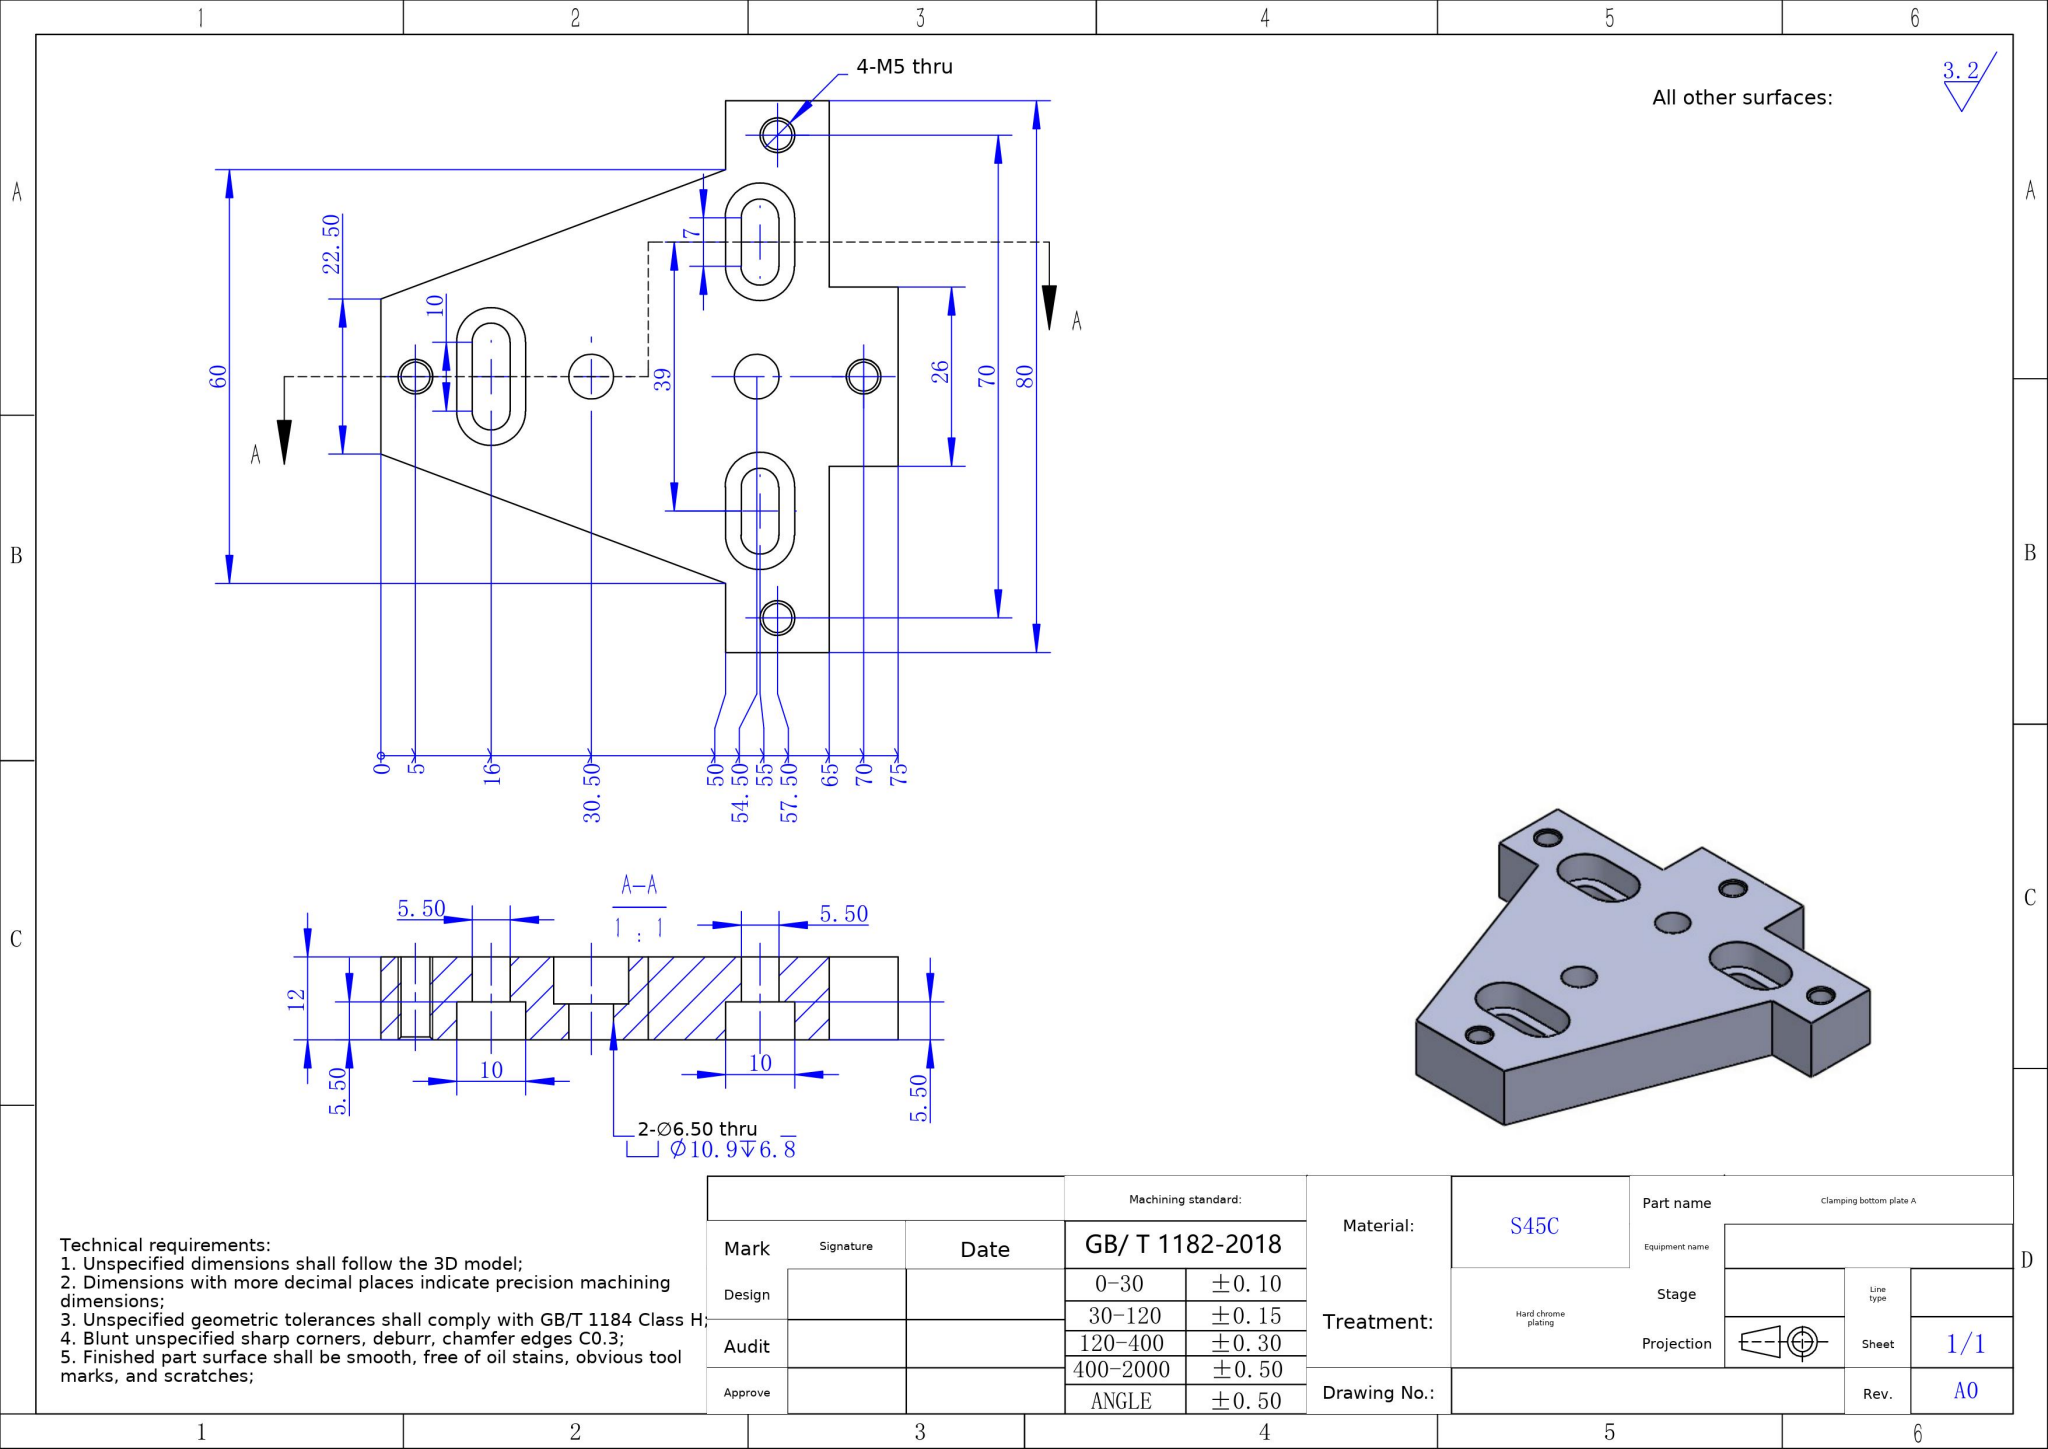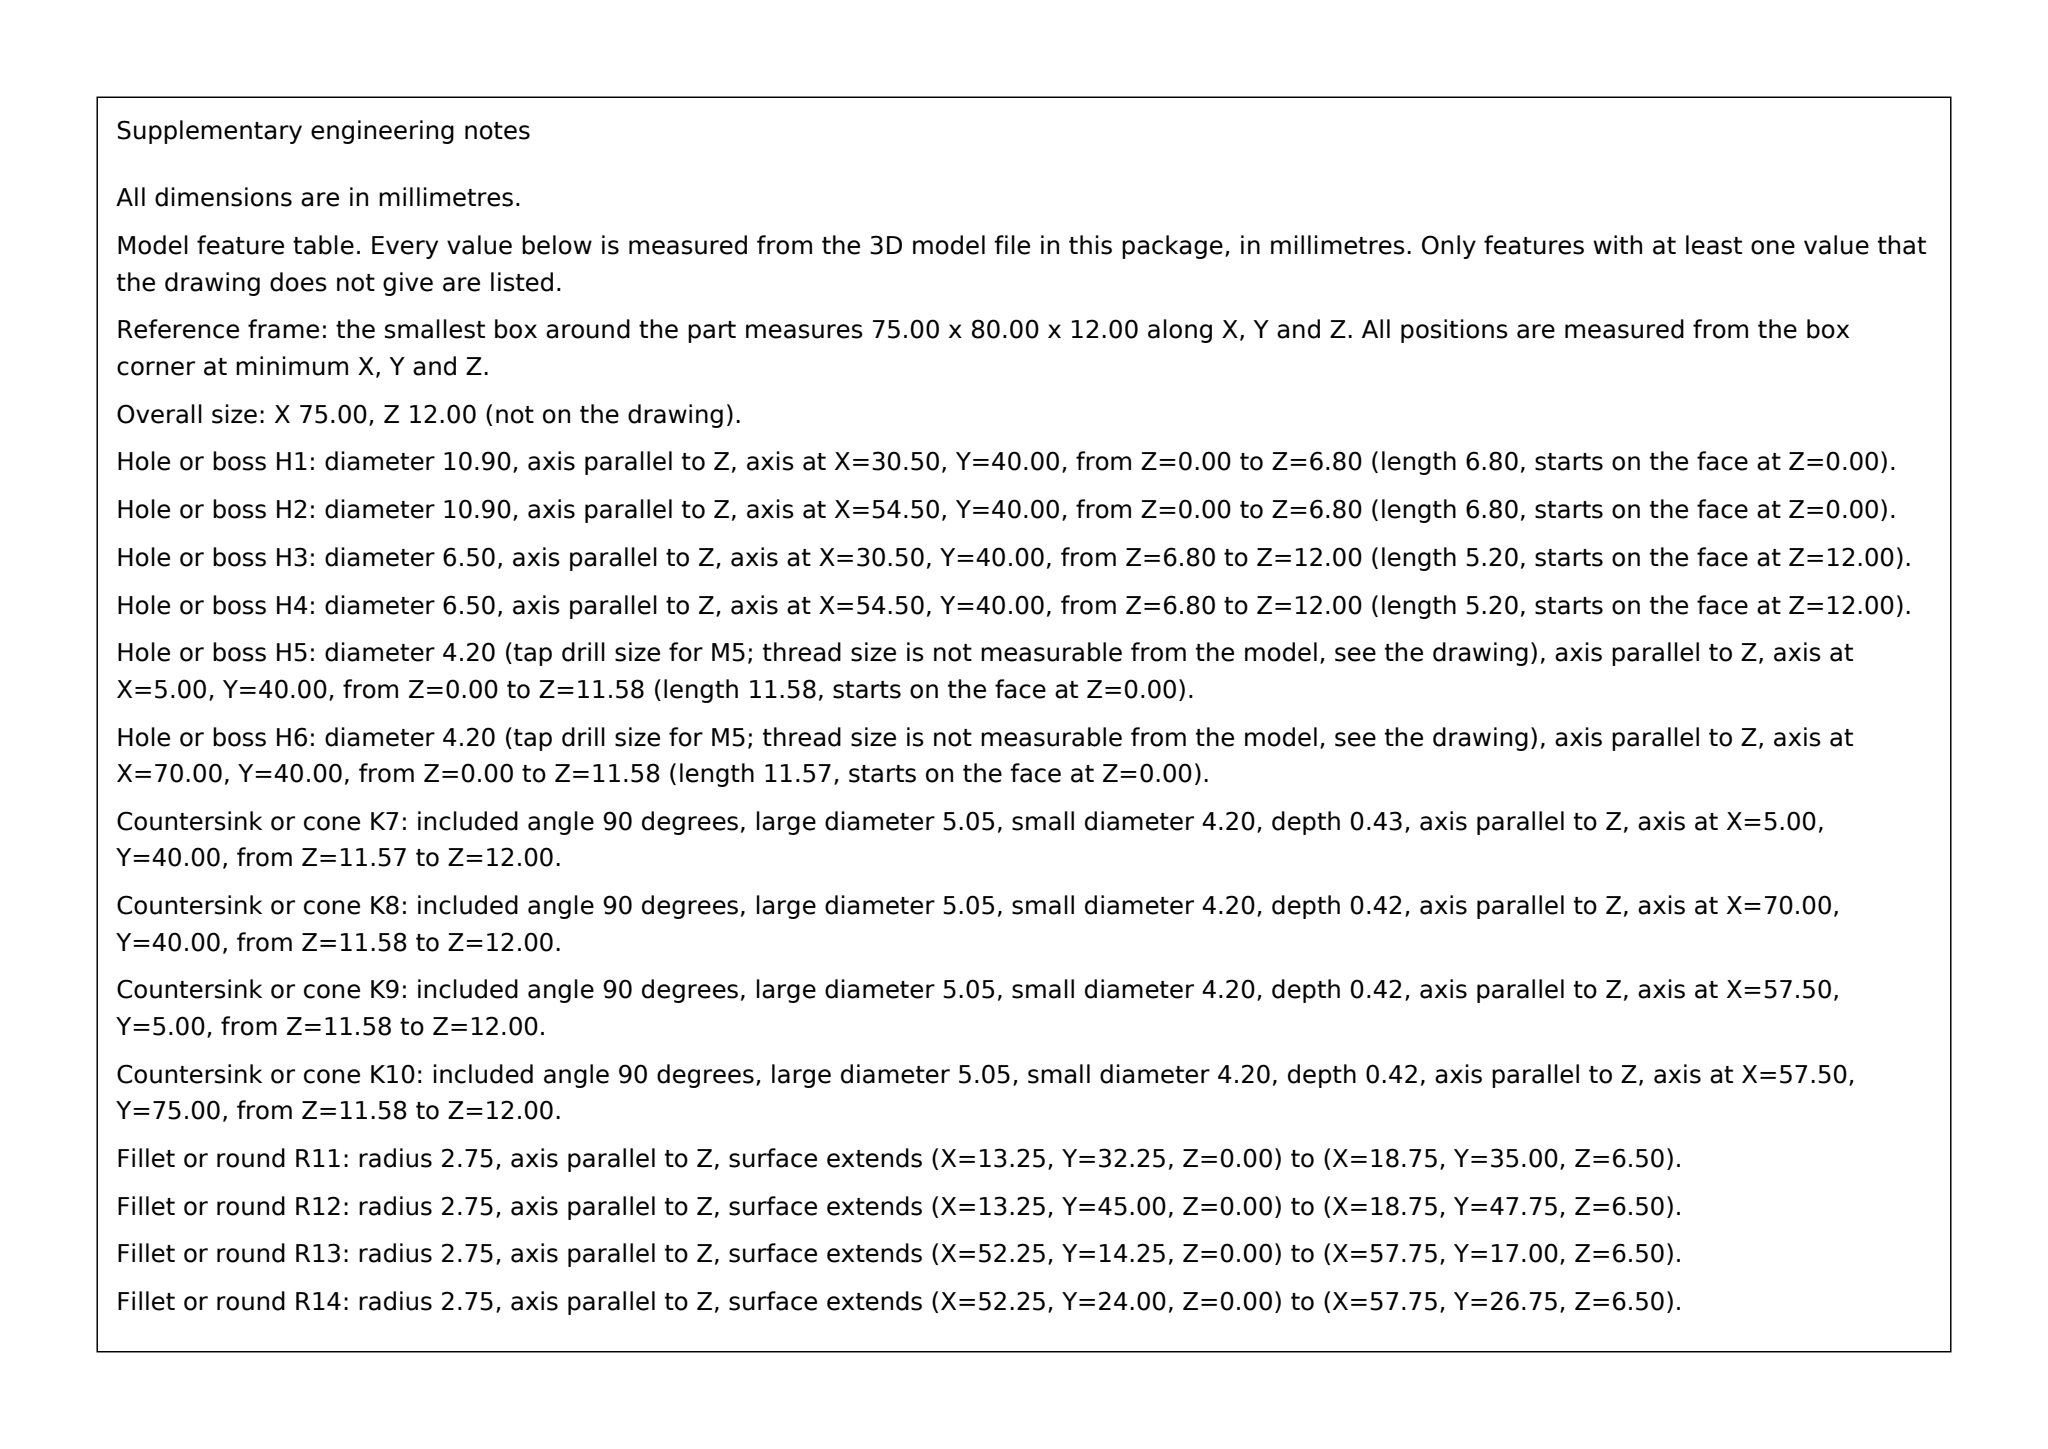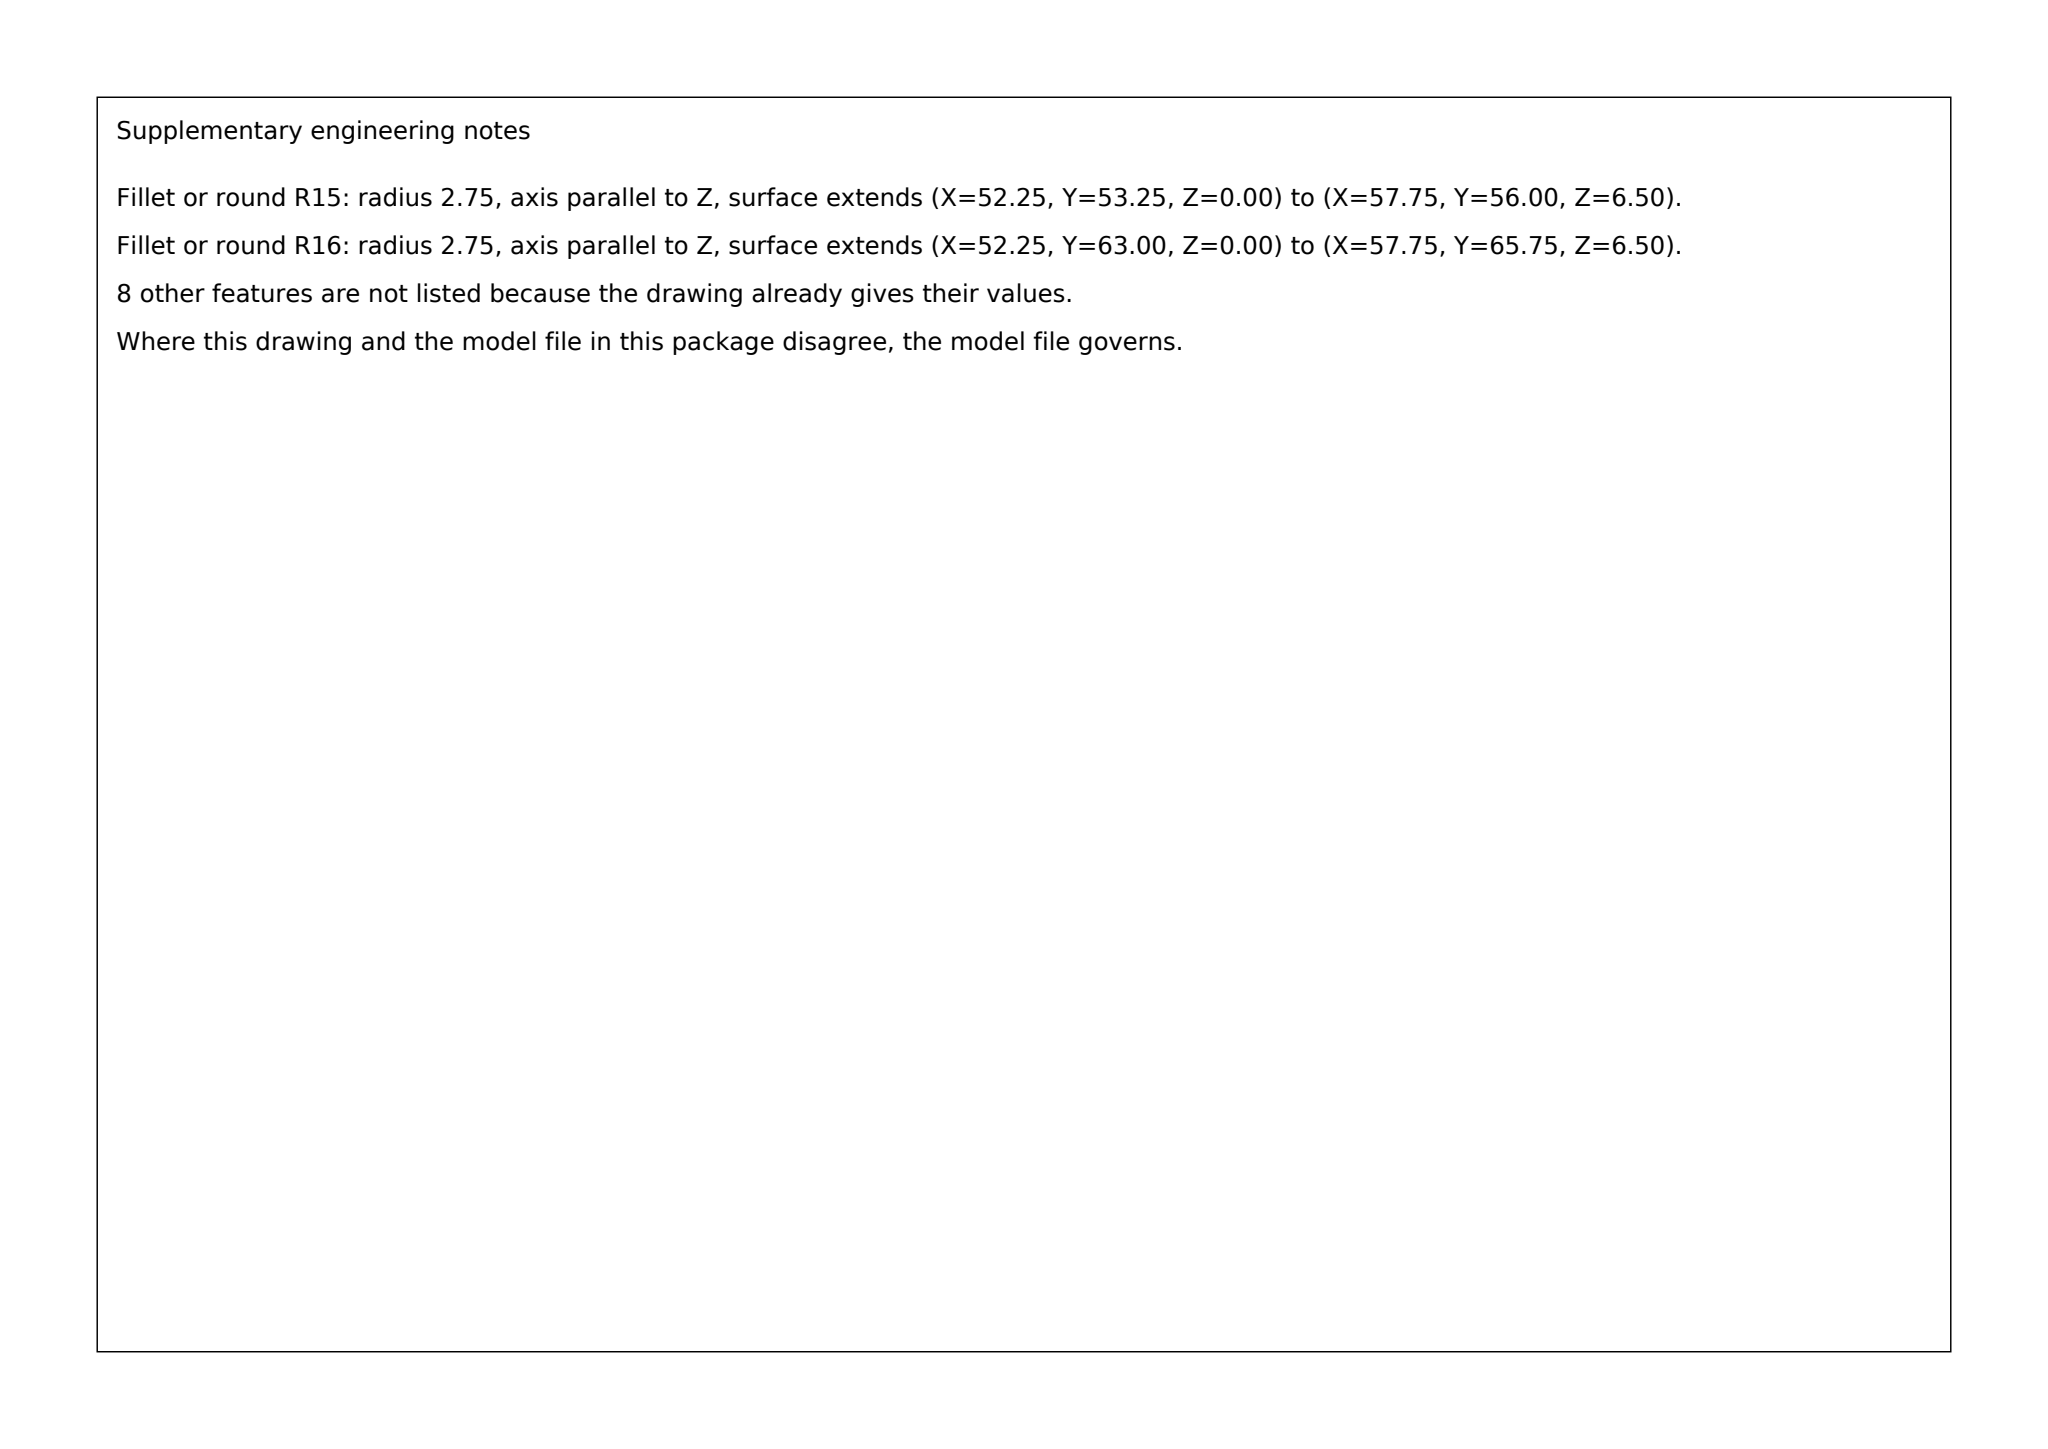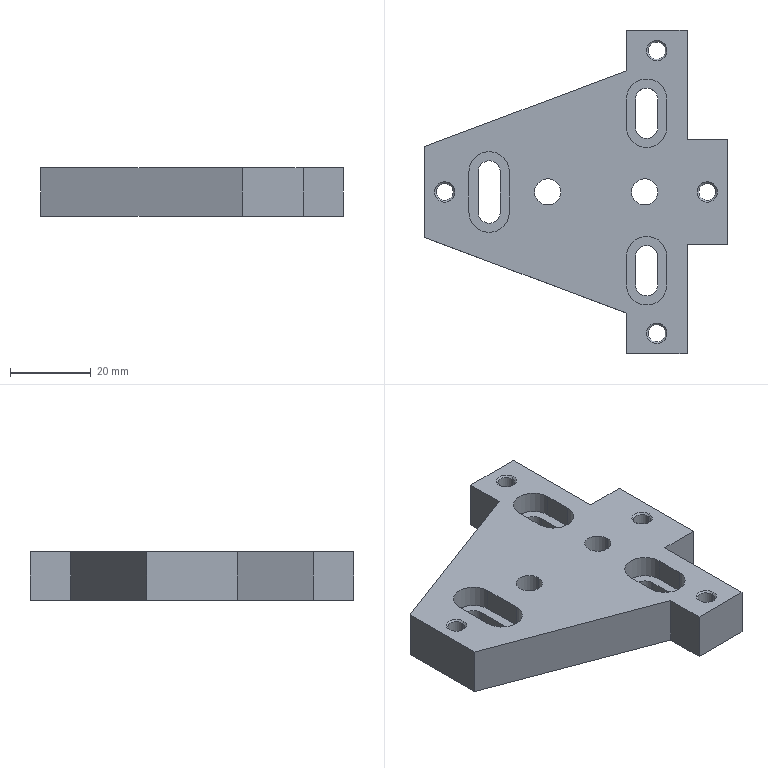Part | SolidWorks | mm | material S45C | 1 solid | 67 faces | box 75 x 80 x 12 mm | volume 36049 mm3 | plane 31 | cylinder 28 | cone 8 | commonest cylinder face diameters 4.2 x8 5.5 x6 10 x6 10.9 x4 6.5 x4
build123d program:
from build123d import *

# Parameters (mm, degrees)
BOSS_EXTRUDE1_DEPTH         = 12
CUT_EXTRUDE1_DEPTH          = 64.789
CUT_EXTRUDE2_DEPTH          = 5.5
SKETCH4_R                   = 3.25
CUT_EXTRUDE3_DEPTH          = 64.789
SKETCH5_W                   = 10
SKETCH5_H                   = 30
SKETCH5_W_2                 = 15
SKETCH5_H_2                 = 10
BOSS_EXTRUDE2_DEPTH         = 12
M5_TAPPED_HOLE1_D           = 4.2
M5_TAPPED_HOLE1_CSINK_D     = 5.05
M5_TAPPED_HOLE1_CSINK_ANGLE = 90
CUT_EXTRUDE4_DEPTH          = 78.259
SKETCH9_W                   = 10
SKETCH9_H                   = 26
BOSS_EXTRUDE3_DEPTH         = 12
M5_TAPPED_HOLE2_D           = 4.2
M5_TAPPED_HOLE2_CSINK_D     = 5.05
M5_TAPPED_HOLE2_CSINK_ANGLE = 90
SKETCH12_R                  = 5.45
CUT_EXTRUDE5_DEPTH          = 6.8


with BuildPart() as part:
    # Sketch1 → Boss-Extrude1 (new body)
    with BuildSketch(Plane.XY):
        Polygon((0, -30), (0, 30), (-15, 30), (-55, 15), (-55, -15), (-15, -30), align=None)
    extrude(amount=BOSS_EXTRUDE1_DEPTH)

    # Sketch2 → Cut-Extrude1 (cut, through all)
    with BuildSketch(Plane.XY.offset(12)):
        with BuildLine():
            Line((-46.25, 5), (-46.25, -5))
            ThreePointArc((-46.25, -5), (-49, -7.75), (-51.75, -5))
            Line((-51.75, -5), (-51.75, 5))
            ThreePointArc((-51.75, 5), (-49, 7.75), (-46.25, 5))
        make_face()
        with BuildLine():
            Line((-7.25, 23), (-7.25, 16))
            ThreePointArc((-7.25, 16), (-10, 13.25), (-12.75, 16))
            Line((-12.75, 16), (-12.75, 23))
            ThreePointArc((-12.75, 23), (-10, 25.75), (-7.25, 23))
        make_face()
        with BuildLine():
            Line((-7.25, -23), (-7.25, -16))
            ThreePointArc((-7.25, -16), (-10, -13.25), (-12.75, -16))
            Line((-12.75, -16), (-12.75, -23))
            ThreePointArc((-12.75, -23), (-10, -25.75), (-7.25, -23))
        make_face()
    extrude(amount=-CUT_EXTRUDE1_DEPTH, mode=Mode.SUBTRACT)

    # Sketch3 → Cut-Extrude2 (cut)
    with BuildSketch(Plane.XY.offset(12)):
        with BuildLine():
            Line((-44, -5), (-44, 5))
            ThreePointArc((-44, 5), (-49, 10), (-54, 5))
            Line((-54, 5), (-54, -5))
            ThreePointArc((-54, -5), (-49, -10), (-44, -5))
        make_face()
        with BuildLine():
            Line((-5, -23), (-5, -16))
            ThreePointArc((-5, -16), (-10, -11), (-15, -16))
            Line((-15, -16), (-15, -23))
            ThreePointArc((-15, -23), (-10, -28), (-5, -23))
        make_face()
        with BuildLine():
            Line((-5, 16), (-5, 23))
            ThreePointArc((-5, 23), (-10, 28), (-15, 23))
            Line((-15, 23), (-15, 16))
            ThreePointArc((-15, 16), (-10, 11), (-5, 16))
        make_face()
    extrude(amount=-CUT_EXTRUDE2_DEPTH, mode=Mode.SUBTRACT)

    # Sketch4 → Cut-Extrude3 (cut, through all)
    with BuildSketch(Plane.XY.offset(12)):
        with Locations((-34.5, 0)):
            Circle(SKETCH4_R)
        with Locations((-10.5, 0)):
            Circle(SKETCH4_R)
    extrude(amount=-CUT_EXTRUDE3_DEPTH, mode=Mode.SUBTRACT)

    # Sketch5 → Boss-Extrude2 (add)
    with BuildSketch(Plane.XY.offset(12)):
        with Locations((-60, 0)):
            Rectangle(SKETCH5_W, SKETCH5_H)
        with Locations((-7.5, 35)):
            Rectangle(SKETCH5_W_2, SKETCH5_H_2)
        with Locations((-7.5, -35)):
            Rectangle(SKETCH5_W_2, SKETCH5_H_2)
    extrude(amount=-BOSS_EXTRUDE2_DEPTH)

    # M5 Tapped Hole1 (through all)
    with Locations(Plane.XY.offset(12)):
        with Locations((-7.5, -35), (-60, 0), (-7.5, 35)):
            CounterSinkHole(M5_TAPPED_HOLE1_D / 2, M5_TAPPED_HOLE1_CSINK_D / 2, counter_sink_angle=M5_TAPPED_HOLE1_CSINK_ANGLE)

    # Sketch8 → Cut-Extrude4 (cut, through all)
    with BuildSketch(Plane.XY.offset(12)):
        Polygon((-55, 15), (-68.605, 22.741), (-66.181, 10.807), align=None)
        Polygon((-68.605, -22.741), (-66.181, -10.807), (-55, -15), align=None)
    extrude(amount=-CUT_EXTRUDE4_DEPTH, mode=Mode.SUBTRACT)

    # Sketch9 → Boss-Extrude3 (add)
    with BuildSketch(Plane.XY.offset(12)):
        with Locations((5, 0)):
            Rectangle(SKETCH9_W, SKETCH9_H)
    extrude(amount=-BOSS_EXTRUDE3_DEPTH)

    # M5 Tapped Hole2 (through all)
    with Locations(Plane.XY.offset(12)):
        with Locations((5, 0)):
            CounterSinkHole(M5_TAPPED_HOLE2_D / 2, M5_TAPPED_HOLE2_CSINK_D / 2, counter_sink_angle=M5_TAPPED_HOLE2_CSINK_ANGLE)

    # Sketch12 → Cut-Extrude5 (cut)
    with BuildSketch(Plane(origin=(0, 0, 0), x_dir=(-1, 0, 0), z_dir=(0, 0, -1))):
        with Locations((10.5, 0)):
            Circle(SKETCH12_R)
        with Locations((34.5, 0)):
            Circle(SKETCH12_R)
    extrude(amount=-CUT_EXTRUDE5_DEPTH, mode=Mode.SUBTRACT)


solid = part.part